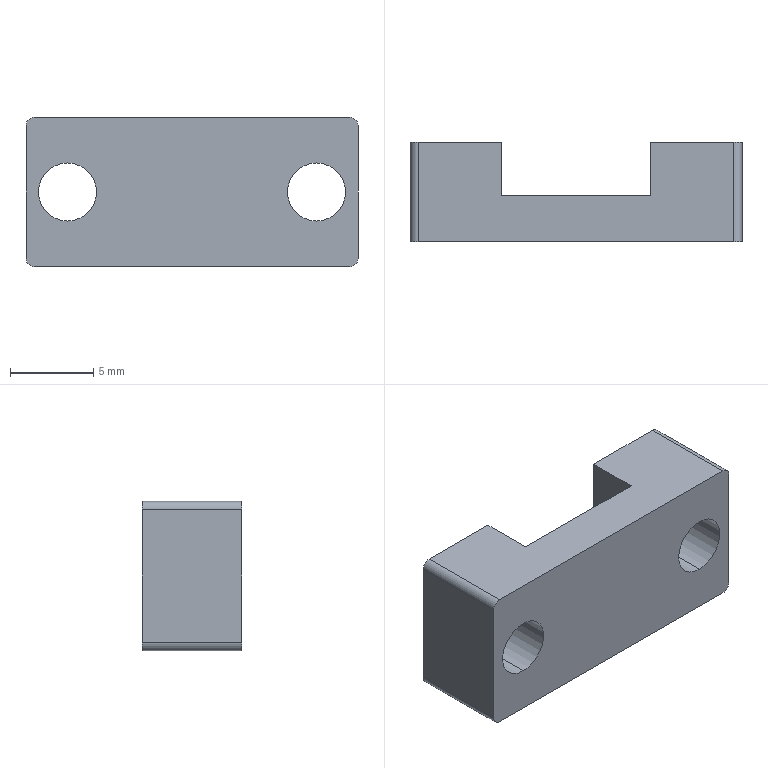Component | SolidWorks | 1ZTJ-NVT-01-011-1-1 | 1 solid | 18 faces | box 20 x 6 x 9 mm | volume 704 mm3 | plane 10 | cylinder 8 | commonest cylinder face diameters 3.5 x4 1 x4 | material #45
build123d program:
from build123d import *

# Parameters (mm, degrees)
SKETCH1_W                      = 20
SKETCH1_H                      = 9
BOSS_EXTRUDE1_DEPTH            = 6
F_3_5_3_5_DIAMETER_HOLE1_D     = 3.5
F_3_5_3_5_DIAMETER_HOLE1_DEPTH = 10
F_3_5_3_5_DIAMETER_HOLE1_TIP   = 1.052
SKETCH15_W                     = 9
SKETCH15_H                     = 3.2
CUT_EXTRUDE1_DEPTH             = 23.738
FILLET5_R                      = 0.5


with BuildPart() as part:
    # Sketch1 → Boss-Extrude1 (new body)
    with BuildSketch(Plane(origin=(0, 0, 0), x_dir=(1, 0, 0), z_dir=(0, 1, 0))):
        with Locations((10, 4.5)):
            Rectangle(SKETCH1_W, SKETCH1_H)
    extrude(amount=BOSS_EXTRUDE1_DEPTH)

    # 3.5 _3.5_ Diameter Hole1
    with Locations(Plane(origin=(0, 6, 0), x_dir=(1, 0, 0), z_dir=(0, 1, 0))):
        with Locations((17.5, 4.5), (2.5, 4.5)):
            Hole(F_3_5_3_5_DIAMETER_HOLE1_D / 2, depth=F_3_5_3_5_DIAMETER_HOLE1_DEPTH)
            with Locations((0, 0, -(F_3_5_3_5_DIAMETER_HOLE1_DEPTH + F_3_5_3_5_DIAMETER_HOLE1_TIP / 2))):  # 118° drill point
                Cone(0, F_3_5_3_5_DIAMETER_HOLE1_D / 2, F_3_5_3_5_DIAMETER_HOLE1_TIP, mode=Mode.SUBTRACT)

    # Sketch15 → Cut-Extrude1 (cut, through all)
    with BuildSketch(Plane(origin=(0, 0, -9), x_dir=(-1, 0, 0), z_dir=(0, 0, -1))):
        with Locations((-10, 4.4)):
            Rectangle(SKETCH15_W, SKETCH15_H)
    extrude(amount=-CUT_EXTRUDE1_DEPTH, mode=Mode.SUBTRACT)

    # Fillet5
    fillet5_edges = [part.edges().sort_by_distance(p)[0] for p in [
        (0, 3, -9),
        (20, 3, -9),
        (20, 3, 0),
        (0, 3, 0),
    ]]
    fillet(fillet5_edges, radius=FILLET5_R)


solid = part.part

# Placed as in the assembly
solid = solid.moved(Location((-23.6, -4.53, 83), (0, 0, 0)))
STEP:
#1=COLOUR_RGB('',0.7922,0.8196,0.9333);
#2=FILL_AREA_STYLE_COLOUR('',#1);
#3=FILL_AREA_STYLE('',(#2));
#4=SURFACE_STYLE_FILL_AREA(#3);
#5=SURFACE_SIDE_STYLE('',(#4));
#6=SURFACE_STYLE_USAGE(.BOTH.,#5);
#7=PRESENTATION_STYLE_ASSIGNMENT((#6));
#8=CARTESIAN_POINT('',(-0.2401,-0.1783,3.159));
#9=VERTEX_POINT('',#8);
#10=CARTESIAN_POINT('',(-0.2401,-0.1783,3.022));
#11=VERTEX_POINT('',#10);
#12=CARTESIAN_POINT('',(-0.2401,-0.1783,3.091));
#13=DIRECTION('',(0.,-1.,0.));
#14=DIRECTION('',(0.,0.,-1.));
#15=AXIS2_PLACEMENT_3D('',#12,#13,#14);
#16=CIRCLE('',#15,0.0689);
#17=EDGE_CURVE('',#9,#11,#16,.T.);
#18=ORIENTED_EDGE('',*,*,#17,.T.);
#19=CARTESIAN_POINT('',(-0.2401,0.05788,3.022));
#20=VERTEX_POINT('',#19);
#21=CARTESIAN_POINT('',(-0.2401,0.05788,3.022));
#22=DIRECTION('',(0.,1.,0.));
#23=VECTOR('',#22,39.37);
#24=LINE('',#21,#23);
#25=EDGE_CURVE('',#11,#20,#24,.T.);
#26=ORIENTED_EDGE('',*,*,#25,.T.);
#27=CARTESIAN_POINT('',(-0.2401,0.05788,3.159));
#28=VERTEX_POINT('',#27);
#29=CARTESIAN_POINT('',(-0.2401,0.05788,3.091));
#30=DIRECTION('',(0.,1.,0.));
#31=DIRECTION('',(0.,0.,1.));
#32=AXIS2_PLACEMENT_3D('',#29,#30,#31);
#33=CIRCLE('',#32,0.0689);
#34=EDGE_CURVE('',#20,#28,#33,.T.);
#35=ORIENTED_EDGE('',*,*,#34,.T.);
#36=CARTESIAN_POINT('',(-0.2401,0.05788,3.159));
#37=DIRECTION('',(0.,1.,0.));
#38=VECTOR('',#37,39.37);
#39=LINE('',#36,#38);
#40=EDGE_CURVE('',#9,#28,#39,.T.);
#41=ORIENTED_EDGE('',*,*,#40,.F.);
#42=EDGE_LOOP('',(#18,#26,#35,#41));
#43=FACE_OUTER_BOUND('',#42,.T.);
#44=CARTESIAN_POINT('',(-0.2401,0.05788,3.091));
#45=DIRECTION('',(0.,1.,0.));
#46=DIRECTION('',(0.,0.,1.));
#47=AXIS2_PLACEMENT_3D('',#44,#45,#46);
#48=CYLINDRICAL_SURFACE('',#47,0.0689);
#49=ADVANCED_FACE('',(#43),#48,.F.);
#50=CARTESIAN_POINT('',(-0.8307,-0.1783,3.159));
#51=VERTEX_POINT('',#50);
#52=CARTESIAN_POINT('',(-0.8307,-0.1783,3.022));
#53=VERTEX_POINT('',#52);
#54=CARTESIAN_POINT('',(-0.8307,-0.1783,3.091));
#55=DIRECTION('',(0.,-1.,0.));
#56=DIRECTION('',(0.,0.,-1.));
#57=AXIS2_PLACEMENT_3D('',#54,#55,#56);
#58=CIRCLE('',#57,0.0689);
#59=EDGE_CURVE('',#51,#53,#58,.T.);
#60=ORIENTED_EDGE('',*,*,#59,.T.);
#61=CARTESIAN_POINT('',(-0.8307,0.05788,3.022));
#62=VERTEX_POINT('',#61);
#63=CARTESIAN_POINT('',(-0.8307,0.05788,3.022));
#64=DIRECTION('',(0.,1.,0.));
#65=VECTOR('',#64,39.37);
#66=LINE('',#63,#65);
#67=EDGE_CURVE('',#53,#62,#66,.T.);
#68=ORIENTED_EDGE('',*,*,#67,.T.);
#69=CARTESIAN_POINT('',(-0.8307,0.05788,3.159));
#70=VERTEX_POINT('',#69);
#71=CARTESIAN_POINT('',(-0.8307,0.05788,3.091));
#72=DIRECTION('',(0.,1.,0.));
#73=DIRECTION('',(0.,0.,1.));
#74=AXIS2_PLACEMENT_3D('',#71,#72,#73);
#75=CIRCLE('',#74,0.0689);
#76=EDGE_CURVE('',#62,#70,#75,.T.);
#77=ORIENTED_EDGE('',*,*,#76,.T.);
#78=CARTESIAN_POINT('',(-0.8307,0.05788,3.159));
#79=DIRECTION('',(0.,1.,0.));
#80=VECTOR('',#79,39.37);
#81=LINE('',#78,#80);
#82=EDGE_CURVE('',#51,#70,#81,.T.);
#83=ORIENTED_EDGE('',*,*,#82,.F.);
#84=EDGE_LOOP('',(#60,#68,#77,#83));
#85=FACE_OUTER_BOUND('',#84,.T.);
#86=CARTESIAN_POINT('',(-0.8307,0.05788,3.091));
#87=DIRECTION('',(0.,1.,0.));
#88=DIRECTION('',(0.,0.,1.));
#89=AXIS2_PLACEMENT_3D('',#86,#87,#88);
#90=CYLINDRICAL_SURFACE('',#89,0.0689);
#91=ADVANCED_FACE('',(#85),#90,.F.);
#92=CARTESIAN_POINT('',(-0.2401,0.05788,3.091));
#93=DIRECTION('',(0.,1.,0.));
#94=DIRECTION('',(0.,0.,1.));
#95=AXIS2_PLACEMENT_3D('',#92,#93,#94);
#96=CIRCLE('',#95,0.0689);
#97=EDGE_CURVE('',#28,#20,#96,.T.);
#98=ORIENTED_EDGE('',*,*,#97,.F.);
#99=ORIENTED_EDGE('',*,*,#34,.F.);
#100=EDGE_LOOP('',(#98,#99));
#101=FACE_BOUND('',#100,.T.);
#102=CARTESIAN_POINT('',(-0.3583,0.05788,3.268));
#103=VERTEX_POINT('',#102);
#104=CARTESIAN_POINT('',(-0.1614,0.05788,3.268));
#105=VERTEX_POINT('',#104);
#106=CARTESIAN_POINT('',(-0.9291,0.05788,3.268));
#107=DIRECTION('',(1.,0.,0.));
#108=VECTOR('',#107,39.37);
#109=LINE('',#106,#108);
#110=EDGE_CURVE('',#103,#105,#109,.T.);
#111=ORIENTED_EDGE('',*,*,#110,.T.);
#112=CARTESIAN_POINT('',(-0.1417,0.05788,3.248));
#113=VERTEX_POINT('',#112);
#114=CARTESIAN_POINT('',(-0.1614,0.05788,3.248));
#115=DIRECTION('',(0.,1.,0.));
#116=DIRECTION('',(0.,0.,-1.));
#117=AXIS2_PLACEMENT_3D('',#114,#115,#116);
#118=CIRCLE('',#117,0.01969);
#119=EDGE_CURVE('',#105,#113,#118,.T.);
#120=ORIENTED_EDGE('',*,*,#119,.T.);
#121=CARTESIAN_POINT('',(-0.1417,0.05788,2.933));
#122=VERTEX_POINT('',#121);
#123=CARTESIAN_POINT('',(-0.1417,0.05788,3.268));
#124=DIRECTION('',(0.,0.,-1.));
#125=VECTOR('',#124,39.37);
#126=LINE('',#123,#125);
#127=EDGE_CURVE('',#113,#122,#126,.T.);
#128=ORIENTED_EDGE('',*,*,#127,.T.);
#129=CARTESIAN_POINT('',(-0.1614,0.05788,2.913));
#130=VERTEX_POINT('',#129);
#131=CARTESIAN_POINT('',(-0.1614,0.05788,2.933));
#132=DIRECTION('',(0.,1.,0.));
#133=DIRECTION('',(0.,0.,-1.));
#134=AXIS2_PLACEMENT_3D('',#131,#132,#133);
#135=CIRCLE('',#134,0.01969);
#136=EDGE_CURVE('',#122,#130,#135,.T.);
#137=ORIENTED_EDGE('',*,*,#136,.T.);
#138=CARTESIAN_POINT('',(-0.3583,0.05788,2.913));
#139=VERTEX_POINT('',#138);
#140=CARTESIAN_POINT('',(-0.9291,0.05788,2.913));
#141=DIRECTION('',(-1.,0.,0.));
#142=VECTOR('',#141,39.37);
#143=LINE('',#140,#142);
#144=EDGE_CURVE('',#130,#139,#143,.T.);
#145=ORIENTED_EDGE('',*,*,#144,.T.);
#146=CARTESIAN_POINT('',(-0.3583,0.05788,3.268));
#147=DIRECTION('',(0.,0.,-1.));
#148=VECTOR('',#147,39.37);
#149=LINE('',#146,#148);
#150=EDGE_CURVE('',#103,#139,#149,.T.);
#151=ORIENTED_EDGE('',*,*,#150,.F.);
#152=EDGE_LOOP('',(#111,#120,#128,#137,#145,#151));
#153=FACE_OUTER_BOUND('',#152,.T.);
#154=CARTESIAN_POINT('',(-0.9291,0.05788,3.268));
#155=DIRECTION('',(0.,-1.,0.));
#156=DIRECTION('',(0.,0.,-1.));
#157=AXIS2_PLACEMENT_3D('',#154,#155,#156);
#158=PLANE('',#157);
#159=ADVANCED_FACE('',(#101,#153),#158,.F.);
#160=CARTESIAN_POINT('',(-0.9291,-0.1783,2.933));
#161=VERTEX_POINT('',#160);
#162=CARTESIAN_POINT('',(-0.9291,-0.1783,3.248));
#163=VERTEX_POINT('',#162);
#164=CARTESIAN_POINT('',(-0.9291,-0.1783,3.268));
#165=DIRECTION('',(0.,0.,1.));
#166=VECTOR('',#165,39.37);
#167=LINE('',#164,#166);
#168=EDGE_CURVE('',#161,#163,#167,.T.);
#169=ORIENTED_EDGE('',*,*,#168,.T.);
#170=CARTESIAN_POINT('',(-0.9291,0.05788,3.248));
#171=VERTEX_POINT('',#170);
#172=CARTESIAN_POINT('',(-0.9291,0.05788,3.248));
#173=DIRECTION('',(0.,1.,0.));
#174=VECTOR('',#173,39.37);
#175=LINE('',#172,#174);
#176=EDGE_CURVE('',#163,#171,#175,.T.);
#177=ORIENTED_EDGE('',*,*,#176,.T.);
#178=CARTESIAN_POINT('',(-0.9291,0.05788,2.933));
#179=VERTEX_POINT('',#178);
#180=CARTESIAN_POINT('',(-0.9291,0.05788,3.268));
#181=DIRECTION('',(0.,0.,1.));
#182=VECTOR('',#181,39.37);
#183=LINE('',#180,#182);
#184=EDGE_CURVE('',#179,#171,#183,.T.);
#185=ORIENTED_EDGE('',*,*,#184,.F.);
#186=CARTESIAN_POINT('',(-0.9291,0.05788,2.933));
#187=DIRECTION('',(0.,-1.,0.));
#188=VECTOR('',#187,39.37);
#189=LINE('',#186,#188);
#190=EDGE_CURVE('',#179,#161,#189,.T.);
#191=ORIENTED_EDGE('',*,*,#190,.T.);
#192=EDGE_LOOP('',(#169,#177,#185,#191));
#193=FACE_OUTER_BOUND('',#192,.T.);
#194=CARTESIAN_POINT('',(-0.9291,0.05788,3.268));
#195=DIRECTION('',(1.,0.,0.));
#196=DIRECTION('',(0.,0.,-1.));
#197=AXIS2_PLACEMENT_3D('',#194,#195,#196);
#198=PLANE('',#197);
#199=ADVANCED_FACE('',(#193),#198,.F.);
#200=CARTESIAN_POINT('',(-0.9094,0.05788,3.268));
#201=VERTEX_POINT('',#200);
#202=CARTESIAN_POINT('',(-0.7126,0.05788,3.268));
#203=VERTEX_POINT('',#202);
#204=CARTESIAN_POINT('',(-0.9291,0.05788,3.268));
#205=DIRECTION('',(1.,0.,0.));
#206=VECTOR('',#205,39.37);
#207=LINE('',#204,#206);
#208=EDGE_CURVE('',#201,#203,#207,.T.);
#209=ORIENTED_EDGE('',*,*,#208,.F.);
#210=CARTESIAN_POINT('',(-0.9094,-0.1783,3.268));
#211=VERTEX_POINT('',#210);
#212=CARTESIAN_POINT('',(-0.9094,0.05788,3.268));
#213=DIRECTION('',(0.,-1.,0.));
#214=VECTOR('',#213,39.37);
#215=LINE('',#212,#214);
#216=EDGE_CURVE('',#201,#211,#215,.T.);
#217=ORIENTED_EDGE('',*,*,#216,.T.);
#218=CARTESIAN_POINT('',(-0.1614,-0.1783,3.268));
#219=VERTEX_POINT('',#218);
#220=CARTESIAN_POINT('',(-0.9291,-0.1783,3.268));
#221=DIRECTION('',(1.,0.,0.));
#222=VECTOR('',#221,39.37);
#223=LINE('',#220,#222);
#224=EDGE_CURVE('',#211,#219,#223,.T.);
#225=ORIENTED_EDGE('',*,*,#224,.T.);
#226=CARTESIAN_POINT('',(-0.1614,0.05788,3.268));
#227=DIRECTION('',(0.,1.,0.));
#228=VECTOR('',#227,39.37);
#229=LINE('',#226,#228);
#230=EDGE_CURVE('',#219,#105,#229,.T.);
#231=ORIENTED_EDGE('',*,*,#230,.T.);
#232=ORIENTED_EDGE('',*,*,#110,.F.);
#233=CARTESIAN_POINT('',(-0.3583,-0.0681,3.268));
#234=VERTEX_POINT('',#233);
#235=CARTESIAN_POINT('',(-0.3583,0.05788,3.268));
#236=DIRECTION('',(0.,-1.,0.));
#237=VECTOR('',#236,39.37);
#238=LINE('',#235,#237);
#239=EDGE_CURVE('',#103,#234,#238,.T.);
#240=ORIENTED_EDGE('',*,*,#239,.T.);
#241=CARTESIAN_POINT('',(-0.7126,-0.0681,3.268));
#242=VERTEX_POINT('',#241);
#243=CARTESIAN_POINT('',(-0.3583,-0.0681,3.268));
#244=DIRECTION('',(-1.,0.,0.));
#245=VECTOR('',#244,39.37);
#246=LINE('',#243,#245);
#247=EDGE_CURVE('',#234,#242,#246,.T.);
#248=ORIENTED_EDGE('',*,*,#247,.T.);
#249=CARTESIAN_POINT('',(-0.7126,0.05788,3.268));
#250=DIRECTION('',(0.,1.,0.));
#251=VECTOR('',#250,39.37);
#252=LINE('',#249,#251);
#253=EDGE_CURVE('',#242,#203,#252,.T.);
#254=ORIENTED_EDGE('',*,*,#253,.T.);
#255=EDGE_LOOP('',(#209,#217,#225,#231,#232,#240,#248,#254));
#256=FACE_OUTER_BOUND('',#255,.T.);
#257=CARTESIAN_POINT('',(-0.9291,0.05788,3.268));
#258=DIRECTION('',(0.,0.,-1.));
#259=DIRECTION('',(-1.,0.,0.));
#260=AXIS2_PLACEMENT_3D('',#257,#258,#259);
#261=PLANE('',#260);
#262=ADVANCED_FACE('',(#256),#261,.F.);
#263=ORIENTED_EDGE('',*,*,#127,.F.);
#264=CARTESIAN_POINT('',(-0.1417,-0.1783,3.248));
#265=VERTEX_POINT('',#264);
#266=CARTESIAN_POINT('',(-0.1417,0.05788,3.248));
#267=DIRECTION('',(0.,-1.,0.));
#268=VECTOR('',#267,39.37);
#269=LINE('',#266,#268);
#270=EDGE_CURVE('',#113,#265,#269,.T.);
#271=ORIENTED_EDGE('',*,*,#270,.T.);
#272=CARTESIAN_POINT('',(-0.1417,-0.1783,2.933));
#273=VERTEX_POINT('',#272);
#274=CARTESIAN_POINT('',(-0.1417,-0.1783,3.268));
#275=DIRECTION('',(0.,0.,-1.));
#276=VECTOR('',#275,39.37);
#277=LINE('',#274,#276);
#278=EDGE_CURVE('',#265,#273,#277,.T.);
#279=ORIENTED_EDGE('',*,*,#278,.T.);
#280=CARTESIAN_POINT('',(-0.1417,0.05788,2.933));
#281=DIRECTION('',(0.,1.,0.));
#282=VECTOR('',#281,39.37);
#283=LINE('',#280,#282);
#284=EDGE_CURVE('',#273,#122,#283,.T.);
#285=ORIENTED_EDGE('',*,*,#284,.T.);
#286=EDGE_LOOP('',(#263,#271,#279,#285));
#287=FACE_OUTER_BOUND('',#286,.T.);
#288=CARTESIAN_POINT('',(-0.1417,0.05788,3.268));
#289=DIRECTION('',(-1.,0.,0.));
#290=DIRECTION('',(0.,0.,1.));
#291=AXIS2_PLACEMENT_3D('',#288,#289,#290);
#292=PLANE('',#291);
#293=ADVANCED_FACE('',(#287),#292,.F.);
#294=CARTESIAN_POINT('',(-0.1614,-0.1783,2.913));
#295=VERTEX_POINT('',#294);
#296=CARTESIAN_POINT('',(-0.9094,-0.1783,2.913));
#297=VERTEX_POINT('',#296);
#298=CARTESIAN_POINT('',(-0.9291,-0.1783,2.913));
#299=DIRECTION('',(-1.,0.,0.));
#300=VECTOR('',#299,39.37);
#301=LINE('',#298,#300);
#302=EDGE_CURVE('',#295,#297,#301,.T.);
#303=ORIENTED_EDGE('',*,*,#302,.T.);
#304=CARTESIAN_POINT('',(-0.9094,0.05788,2.913));
#305=VERTEX_POINT('',#304);
#306=CARTESIAN_POINT('',(-0.9094,0.05788,2.913));
#307=DIRECTION('',(0.,1.,0.));
#308=VECTOR('',#307,39.37);
#309=LINE('',#306,#308);
#310=EDGE_CURVE('',#297,#305,#309,.T.);
#311=ORIENTED_EDGE('',*,*,#310,.T.);
#312=CARTESIAN_POINT('',(-0.7126,0.05788,2.913));
#313=VERTEX_POINT('',#312);
#314=CARTESIAN_POINT('',(-0.9291,0.05788,2.913));
#315=DIRECTION('',(-1.,0.,0.));
#316=VECTOR('',#315,39.37);
#317=LINE('',#314,#316);
#318=EDGE_CURVE('',#313,#305,#317,.T.);
#319=ORIENTED_EDGE('',*,*,#318,.F.);
#320=CARTESIAN_POINT('',(-0.7126,-0.0681,2.913));
#321=VERTEX_POINT('',#320);
#322=CARTESIAN_POINT('',(-0.7126,0.05788,2.913));
#323=DIRECTION('',(0.,1.,0.));
#324=VECTOR('',#323,39.37);
#325=LINE('',#322,#324);
#326=EDGE_CURVE('',#321,#313,#325,.T.);
#327=ORIENTED_EDGE('',*,*,#326,.F.);
#328=CARTESIAN_POINT('',(-0.3583,-0.0681,2.913));
#329=VERTEX_POINT('',#328);
#330=CARTESIAN_POINT('',(-0.3583,-0.0681,2.913));
#331=DIRECTION('',(-1.,0.,0.));
#332=VECTOR('',#331,39.37);
#333=LINE('',#330,#332);
#334=EDGE_CURVE('',#329,#321,#333,.T.);
#335=ORIENTED_EDGE('',*,*,#334,.F.);
#336=CARTESIAN_POINT('',(-0.3583,0.05788,2.913));
#337=DIRECTION('',(0.,-1.,0.));
#338=VECTOR('',#337,39.37);
#339=LINE('',#336,#338);
#340=EDGE_CURVE('',#139,#329,#339,.T.);
#341=ORIENTED_EDGE('',*,*,#340,.F.);
#342=ORIENTED_EDGE('',*,*,#144,.F.);
#343=CARTESIAN_POINT('',(-0.1614,0.05788,2.913));
#344=DIRECTION('',(0.,-1.,0.));
#345=VECTOR('',#344,39.37);
#346=LINE('',#343,#345);
#347=EDGE_CURVE('',#130,#295,#346,.T.);
#348=ORIENTED_EDGE('',*,*,#347,.T.);
#349=EDGE_LOOP('',(#303,#311,#319,#327,#335,#341,#342,#348));
#350=FACE_OUTER_BOUND('',#349,.T.);
#351=CARTESIAN_POINT('',(-0.9291,0.05788,2.913));
#352=DIRECTION('',(0.,0.,1.));
#353=DIRECTION('',(1.,0.,0.));
#354=AXIS2_PLACEMENT_3D('',#351,#352,#353);
#355=PLANE('',#354);
#356=ADVANCED_FACE('',(#350),#355,.F.);
#357=CARTESIAN_POINT('',(-0.8307,0.05788,3.091));
#358=DIRECTION('',(0.,1.,0.));
#359=DIRECTION('',(0.,0.,1.));
#360=AXIS2_PLACEMENT_3D('',#357,#358,#359);
#361=CIRCLE('',#360,0.0689);
#362=EDGE_CURVE('',#70,#62,#361,.T.);
#363=ORIENTED_EDGE('',*,*,#362,.F.);
#364=ORIENTED_EDGE('',*,*,#76,.F.);
#365=EDGE_LOOP('',(#363,#364));
#366=FACE_BOUND('',#365,.T.);
#367=ORIENTED_EDGE('',*,*,#184,.T.);
#368=CARTESIAN_POINT('',(-0.9094,0.05788,3.248));
#369=DIRECTION('',(0.,1.,0.));
#370=DIRECTION('',(0.,0.,-1.));
#371=AXIS2_PLACEMENT_3D('',#368,#369,#370);
#372=CIRCLE('',#371,0.01969);
#373=EDGE_CURVE('',#171,#201,#372,.T.);
#374=ORIENTED_EDGE('',*,*,#373,.T.);
#375=ORIENTED_EDGE('',*,*,#208,.T.);
#376=CARTESIAN_POINT('',(-0.7126,0.05788,3.268));
#377=DIRECTION('',(0.,0.,-1.));
#378=VECTOR('',#377,39.37);
#379=LINE('',#376,#378);
#380=EDGE_CURVE('',#203,#313,#379,.T.);
#381=ORIENTED_EDGE('',*,*,#380,.T.);
#382=ORIENTED_EDGE('',*,*,#318,.T.);
#383=CARTESIAN_POINT('',(-0.9094,0.05788,2.933));
#384=DIRECTION('',(0.,1.,0.));
#385=DIRECTION('',(0.,0.,-1.));
#386=AXIS2_PLACEMENT_3D('',#383,#384,#385);
#387=CIRCLE('',#386,0.01969);
#388=EDGE_CURVE('',#305,#179,#387,.T.);
#389=ORIENTED_EDGE('',*,*,#388,.T.);
#390=EDGE_LOOP('',(#367,#374,#375,#381,#382,#389));
#391=FACE_OUTER_BOUND('',#390,.T.);
#392=CARTESIAN_POINT('',(-0.9291,0.05788,3.268));
#393=DIRECTION('',(0.,-1.,0.));
#394=DIRECTION('',(0.,0.,-1.));
#395=AXIS2_PLACEMENT_3D('',#392,#393,#394);
#396=PLANE('',#395);
#397=ADVANCED_FACE('',(#366,#391),#396,.F.);
#398=ORIENTED_EDGE('',*,*,#17,.F.);
#399=CARTESIAN_POINT('',(-0.2401,-0.1783,3.091));
#400=DIRECTION('',(0.,-1.,0.));
#401=DIRECTION('',(0.,0.,-1.));
#402=AXIS2_PLACEMENT_3D('',#399,#400,#401);
#403=CIRCLE('',#402,0.0689);
#404=EDGE_CURVE('',#11,#9,#403,.T.);
#405=ORIENTED_EDGE('',*,*,#404,.F.);
#406=EDGE_LOOP('',(#398,#405));
#407=FACE_BOUND('',#406,.T.);
#408=ORIENTED_EDGE('',*,*,#59,.F.);
#409=CARTESIAN_POINT('',(-0.8307,-0.1783,3.091));
#410=DIRECTION('',(0.,-1.,0.));
#411=DIRECTION('',(0.,0.,-1.));
#412=AXIS2_PLACEMENT_3D('',#409,#410,#411);
#413=CIRCLE('',#412,0.0689);
#414=EDGE_CURVE('',#53,#51,#413,.T.);
#415=ORIENTED_EDGE('',*,*,#414,.F.);
#416=EDGE_LOOP('',(#408,#415));
#417=FACE_BOUND('',#416,.T.);
#418=ORIENTED_EDGE('',*,*,#224,.F.);
#419=CARTESIAN_POINT('',(-0.9094,-0.1783,3.248));
#420=DIRECTION('',(0.,-1.,0.));
#421=DIRECTION('',(0.,0.,-1.));
#422=AXIS2_PLACEMENT_3D('',#419,#420,#421);
#423=CIRCLE('',#422,0.01969);
#424=EDGE_CURVE('',#211,#163,#423,.T.);
#425=ORIENTED_EDGE('',*,*,#424,.T.);
#426=ORIENTED_EDGE('',*,*,#168,.F.);
#427=CARTESIAN_POINT('',(-0.9094,-0.1783,2.933));
#428=DIRECTION('',(0.,-1.,0.));
#429=DIRECTION('',(0.,0.,-1.));
#430=AXIS2_PLACEMENT_3D('',#427,#428,#429);
#431=CIRCLE('',#430,0.01969);
#432=EDGE_CURVE('',#161,#297,#431,.T.);
#433=ORIENTED_EDGE('',*,*,#432,.T.);
#434=ORIENTED_EDGE('',*,*,#302,.F.);
#435=CARTESIAN_POINT('',(-0.1614,-0.1783,2.933));
#436=DIRECTION('',(0.,-1.,0.));
#437=DIRECTION('',(0.,0.,-1.));
#438=AXIS2_PLACEMENT_3D('',#435,#436,#437);
#439=CIRCLE('',#438,0.01969);
#440=EDGE_CURVE('',#295,#273,#439,.T.);
#441=ORIENTED_EDGE('',*,*,#440,.T.);
#442=ORIENTED_EDGE('',*,*,#278,.F.);
#443=CARTESIAN_POINT('',(-0.1614,-0.1783,3.248));
#444=DIRECTION('',(0.,-1.,0.));
#445=DIRECTION('',(0.,0.,-1.));
#446=AXIS2_PLACEMENT_3D('',#443,#444,#445);
#447=CIRCLE('',#446,0.01969);
#448=EDGE_CURVE('',#265,#219,#447,.T.);
#449=ORIENTED_EDGE('',*,*,#448,.T.);
#450=EDGE_LOOP('',(#418,#425,#426,#433,#434,#441,#442,#449));
#451=FACE_OUTER_BOUND('',#450,.T.);
#452=CARTESIAN_POINT('',(-0.9291,-0.1783,3.268));
#453=DIRECTION('',(0.,-1.,0.));
#454=DIRECTION('',(0.,0.,-1.));
#455=AXIS2_PLACEMENT_3D('',#452,#453,#454);
#456=PLANE('',#455);
#457=ADVANCED_FACE('',(#407,#417,#451),#456,.T.);
#458=ORIENTED_EDGE('',*,*,#67,.F.);
#459=ORIENTED_EDGE('',*,*,#414,.T.);
#460=ORIENTED_EDGE('',*,*,#82,.T.);
#461=ORIENTED_EDGE('',*,*,#362,.T.);
#462=EDGE_LOOP('',(#458,#459,#460,#461));
#463=FACE_OUTER_BOUND('',#462,.T.);
#464=CARTESIAN_POINT('',(-0.8307,0.05788,3.091));
#465=DIRECTION('',(0.,1.,0.));
#466=DIRECTION('',(0.,0.,1.));
#467=AXIS2_PLACEMENT_3D('',#464,#465,#466);
#468=CYLINDRICAL_SURFACE('',#467,0.0689);
#469=ADVANCED_FACE('',(#463),#468,.F.);
#470=ORIENTED_EDGE('',*,*,#25,.F.);
#471=ORIENTED_EDGE('',*,*,#404,.T.);
#472=ORIENTED_EDGE('',*,*,#40,.T.);
#473=ORIENTED_EDGE('',*,*,#97,.T.);
#474=EDGE_LOOP('',(#470,#471,#472,#473));
#475=FACE_OUTER_BOUND('',#474,.T.);
#476=CARTESIAN_POINT('',(-0.2401,0.05788,3.091));
#477=DIRECTION('',(0.,1.,0.));
#478=DIRECTION('',(0.,0.,1.));
#479=AXIS2_PLACEMENT_3D('',#476,#477,#478);
#480=CYLINDRICAL_SURFACE('',#479,0.0689);
#481=ADVANCED_FACE('',(#475),#480,.F.);
#482=ORIENTED_EDGE('',*,*,#340,.T.);
#483=CARTESIAN_POINT('',(-0.3583,-0.0681,3.268));
#484=DIRECTION('',(0.,0.,-1.));
#485=VECTOR('',#484,39.37);
#486=LINE('',#483,#485);
#487=EDGE_CURVE('',#234,#329,#486,.T.);
#488=ORIENTED_EDGE('',*,*,#487,.F.);
#489=ORIENTED_EDGE('',*,*,#239,.F.);
#490=ORIENTED_EDGE('',*,*,#150,.T.);
#491=EDGE_LOOP('',(#482,#488,#489,#490));
#492=FACE_OUTER_BOUND('',#491,.T.);
#493=CARTESIAN_POINT('',(-0.3583,0.05788,3.268));
#494=DIRECTION('',(1.,0.,0.));
#495=DIRECTION('',(0.,0.,-1.));
#496=AXIS2_PLACEMENT_3D('',#493,#494,#495);
#497=PLANE('',#496);
#498=ADVANCED_FACE('',(#492),#497,.F.);
#499=ORIENTED_EDGE('',*,*,#326,.T.);
#500=ORIENTED_EDGE('',*,*,#380,.F.);
#501=ORIENTED_EDGE('',*,*,#253,.F.);
#502=CARTESIAN_POINT('',(-0.7126,-0.0681,3.268));
#503=DIRECTION('',(0.,0.,-1.));
#504=VECTOR('',#503,39.37);
#505=LINE('',#502,#504);
#506=EDGE_CURVE('',#242,#321,#505,.T.);
#507=ORIENTED_EDGE('',*,*,#506,.T.);
#508=EDGE_LOOP('',(#499,#500,#501,#507));
#509=FACE_OUTER_BOUND('',#508,.T.);
#510=CARTESIAN_POINT('',(-0.7126,0.05788,3.268));
#511=DIRECTION('',(-1.,0.,0.));
#512=DIRECTION('',(0.,0.,1.));
#513=AXIS2_PLACEMENT_3D('',#510,#511,#512);
#514=PLANE('',#513);
#515=ADVANCED_FACE('',(#509),#514,.F.);
#516=ORIENTED_EDGE('',*,*,#334,.T.);
#517=ORIENTED_EDGE('',*,*,#506,.F.);
#518=ORIENTED_EDGE('',*,*,#247,.F.);
#519=ORIENTED_EDGE('',*,*,#487,.T.);
#520=EDGE_LOOP('',(#516,#517,#518,#519));
#521=FACE_OUTER_BOUND('',#520,.T.);
#522=CARTESIAN_POINT('',(-0.3583,-0.0681,3.268));
#523=DIRECTION('',(-0.,-1.,0.));
#524=DIRECTION('',(1.,-0.,0.));
#525=AXIS2_PLACEMENT_3D('',#522,#523,#524);
#526=PLANE('',#525);
#527=ADVANCED_FACE('',(#521),#526,.F.);
#528=ORIENTED_EDGE('',*,*,#373,.F.);
#529=ORIENTED_EDGE('',*,*,#176,.F.);
#530=ORIENTED_EDGE('',*,*,#424,.F.);
#531=ORIENTED_EDGE('',*,*,#216,.F.);
#532=EDGE_LOOP('',(#528,#529,#530,#531));
#533=FACE_OUTER_BOUND('',#532,.T.);
#534=CARTESIAN_POINT('',(-0.9094,0.05788,3.248));
#535=DIRECTION('',(0.,-1.,0.));
#536=DIRECTION('',(0.,0.,-1.));
#537=AXIS2_PLACEMENT_3D('',#534,#535,#536);
#538=CYLINDRICAL_SURFACE('',#537,0.01969);
#539=ADVANCED_FACE('',(#533),#538,.T.);
#540=ORIENTED_EDGE('',*,*,#388,.F.);
#541=ORIENTED_EDGE('',*,*,#310,.F.);
#542=ORIENTED_EDGE('',*,*,#432,.F.);
#543=ORIENTED_EDGE('',*,*,#190,.F.);
#544=EDGE_LOOP('',(#540,#541,#542,#543));
#545=FACE_OUTER_BOUND('',#544,.T.);
#546=CARTESIAN_POINT('',(-0.9094,0.05788,2.933));
#547=DIRECTION('',(0.,-1.,0.));
#548=DIRECTION('',(0.,0.,-1.));
#549=AXIS2_PLACEMENT_3D('',#546,#547,#548);
#550=CYLINDRICAL_SURFACE('',#549,0.01969);
#551=ADVANCED_FACE('',(#545),#550,.T.);
#552=ORIENTED_EDGE('',*,*,#119,.F.);
#553=ORIENTED_EDGE('',*,*,#230,.F.);
#554=ORIENTED_EDGE('',*,*,#448,.F.);
#555=ORIENTED_EDGE('',*,*,#270,.F.);
#556=EDGE_LOOP('',(#552,#553,#554,#555));
#557=FACE_OUTER_BOUND('',#556,.T.);
#558=CARTESIAN_POINT('',(-0.1614,0.05788,3.248));
#559=DIRECTION('',(0.,-1.,0.));
#560=DIRECTION('',(0.,0.,-1.));
#561=AXIS2_PLACEMENT_3D('',#558,#559,#560);
#562=CYLINDRICAL_SURFACE('',#561,0.01969);
#563=ADVANCED_FACE('',(#557),#562,.T.);
#564=ORIENTED_EDGE('',*,*,#136,.F.);
#565=ORIENTED_EDGE('',*,*,#284,.F.);
#566=ORIENTED_EDGE('',*,*,#440,.F.);
#567=ORIENTED_EDGE('',*,*,#347,.F.);
#568=EDGE_LOOP('',(#564,#565,#566,#567));
#569=FACE_OUTER_BOUND('',#568,.T.);
#570=CARTESIAN_POINT('',(-0.1614,0.05788,2.933));
#571=DIRECTION('',(0.,-1.,0.));
#572=DIRECTION('',(0.,0.,-1.));
#573=AXIS2_PLACEMENT_3D('',#570,#571,#572);
#574=CYLINDRICAL_SURFACE('',#573,0.01969);
#575=ADVANCED_FACE('',(#569),#574,.T.);
#576=CLOSED_SHELL('',(#49,#91,#159,#199,#262,#293,#356,#397,#457,#469,#481,#498,#515,#527,#539,#551,#563,#575));
#577=MANIFOLD_SOLID_BREP('',#576);
#578=STYLED_ITEM('',(#7),#577);
#579=PRESENTATION_LAYER_ASSIGNMENT('','',(#578));
#580=CARTESIAN_POINT('',(0.,0.,0.));
#581=DIRECTION('',(0.,0.,1.));
#582=DIRECTION('',(1.,0.,0.));
#583=AXIS2_PLACEMENT_3D('',#580,#581,#582);
#584=(LENGTH_UNIT()NAMED_UNIT(*)SI_UNIT($,.METRE.));
#585=LENGTH_MEASURE_WITH_UNIT(LENGTH_MEASURE(0.0254),#584);
#586=DIMENSIONAL_EXPONENTS(1.,0.,0.,0.,0.,0.,0.);
#587=(CONVERSION_BASED_UNIT('',#585)LENGTH_UNIT()NAMED_UNIT(#586));
#588=UNCERTAINTY_MEASURE_WITH_UNIT(LENGTH_MEASURE(0.00001),#587,'','');
#589=(NAMED_UNIT(*)PLANE_ANGLE_UNIT()SI_UNIT($,.RADIAN.));
#590=(NAMED_UNIT(*)SI_UNIT($,.STERADIAN.)SOLID_ANGLE_UNIT());
#591=(GEOMETRIC_REPRESENTATION_CONTEXT(3)GLOBAL_UNCERTAINTY_ASSIGNED_CONTEXT((#588))GLOBAL_UNIT_ASSIGNED_CONTEXT((#587,#589,#590))REPRESENTATION_CONTEXT('',''));
#592=ADVANCED_BREP_SHAPE_REPRESENTATION('',(#577,#583),#591);
#593=(LENGTH_UNIT()NAMED_UNIT(*)SI_UNIT($,.METRE.));
#594=LENGTH_MEASURE_WITH_UNIT(LENGTH_MEASURE(0.0254),#593);
#595=DIMENSIONAL_EXPONENTS(1.,0.,0.,0.,0.,0.,0.);
#596=(CONVERSION_BASED_UNIT('',#594)LENGTH_UNIT()NAMED_UNIT(#595));
#597=UNCERTAINTY_MEASURE_WITH_UNIT(LENGTH_MEASURE(0.00001),#596,'','');
#598=(NAMED_UNIT(*)PLANE_ANGLE_UNIT()SI_UNIT($,.RADIAN.));
#599=(NAMED_UNIT(*)SI_UNIT($,.STERADIAN.)SOLID_ANGLE_UNIT());
#600=(GEOMETRIC_REPRESENTATION_CONTEXT(3)GLOBAL_UNCERTAINTY_ASSIGNED_CONTEXT((#597))GLOBAL_UNIT_ASSIGNED_CONTEXT((#596,#598,#599))REPRESENTATION_CONTEXT('',''));
#601=MECHANICAL_DESIGN_GEOMETRIC_PRESENTATION_REPRESENTATION('',(#578),#600);